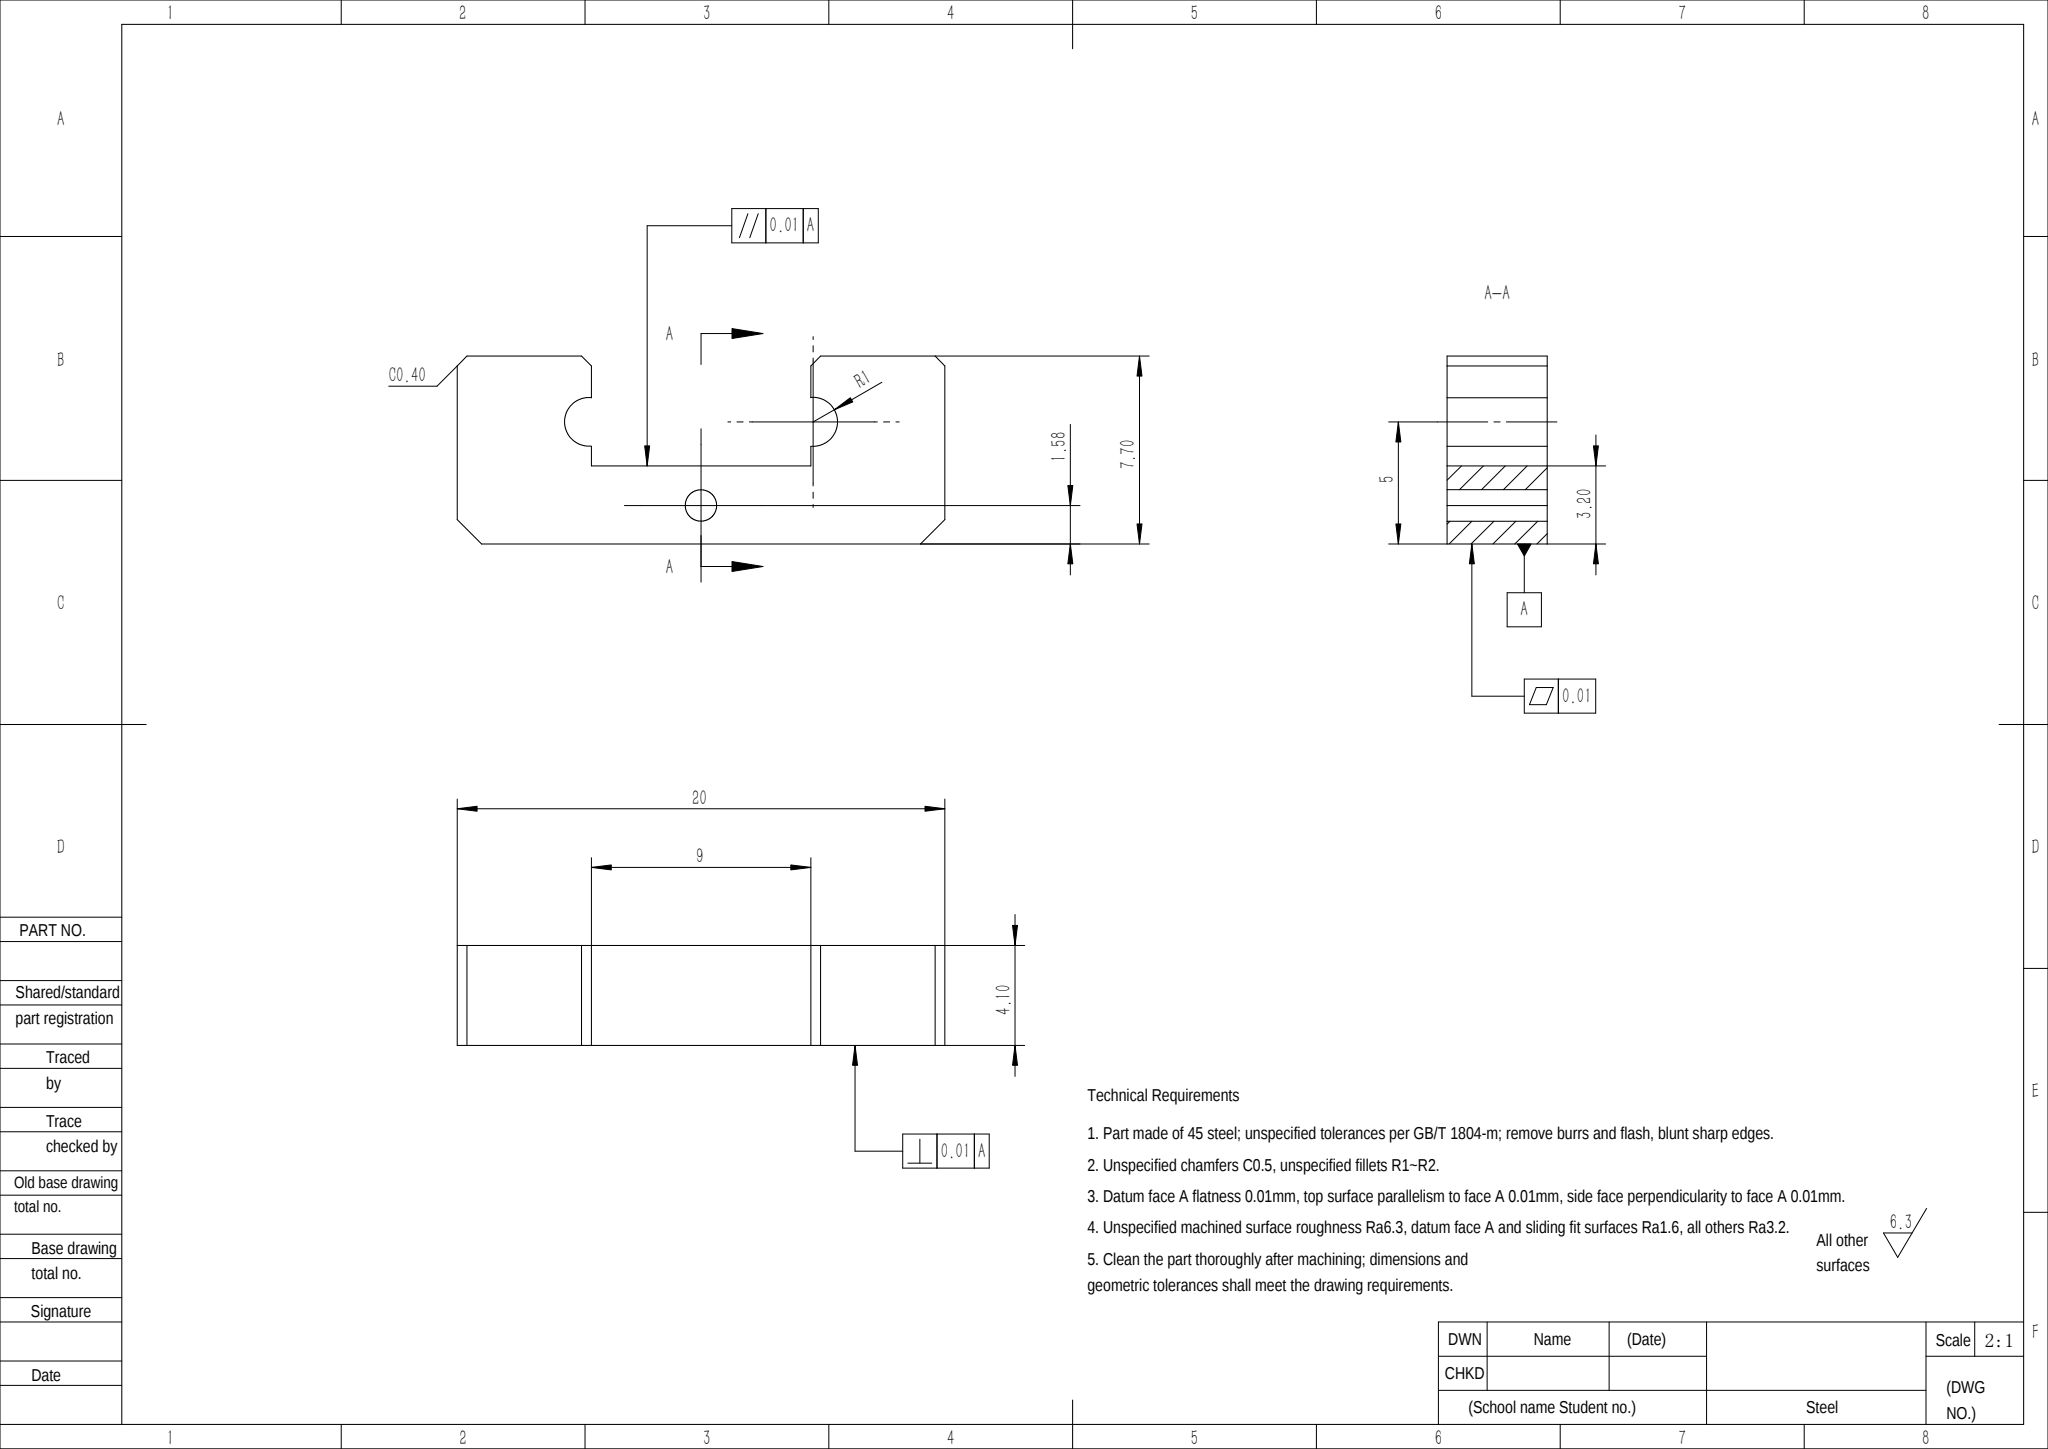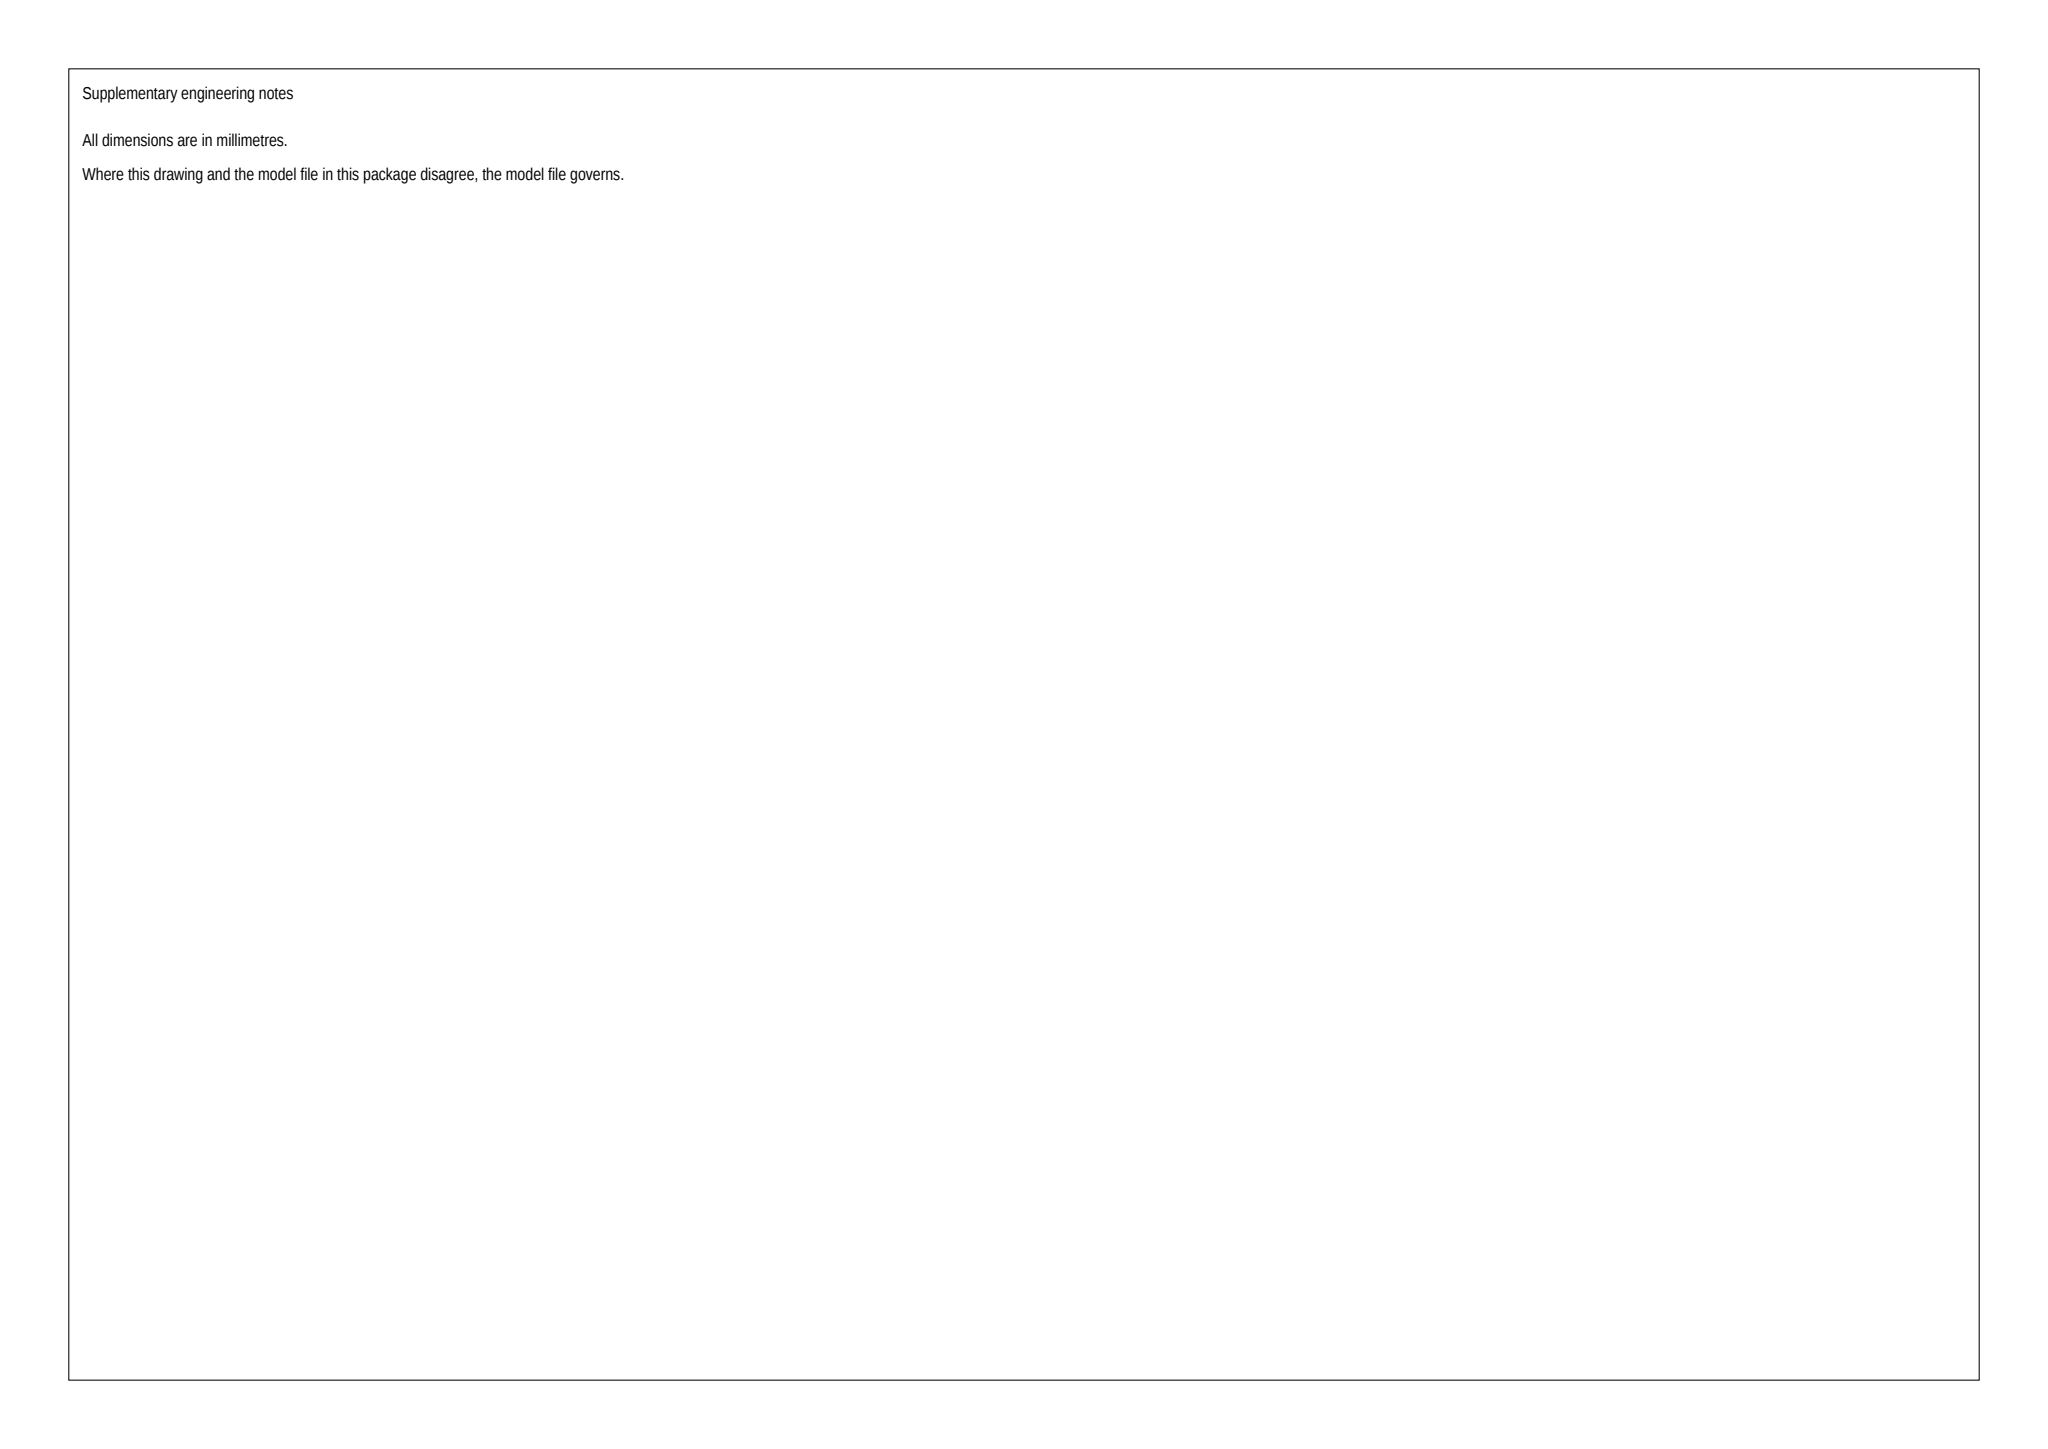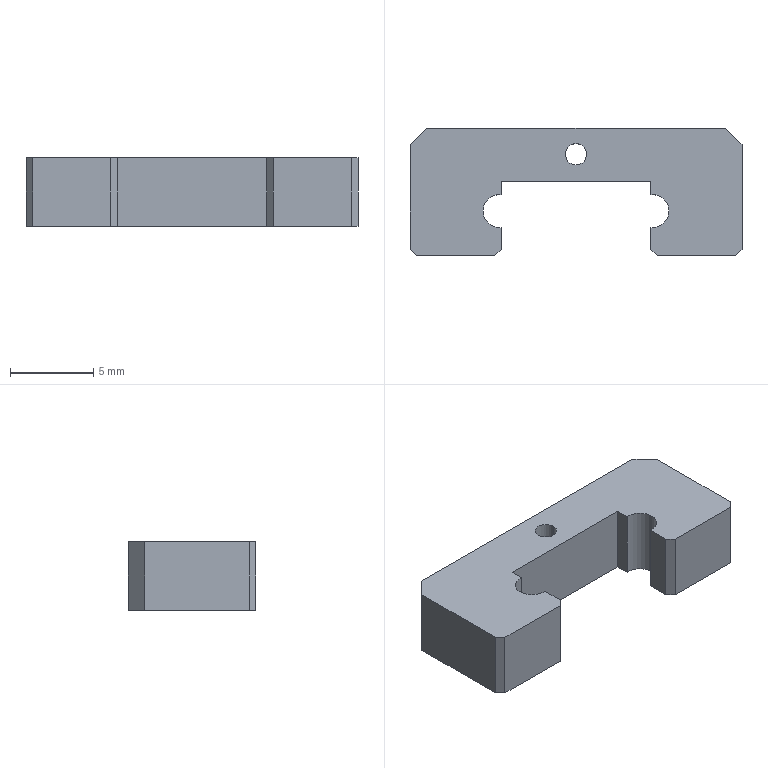Part | SolidWorks | mm | material 45 steel | 1 solid | 22 faces | box 20 x 7.7 x 4.1 mm | volume 440 mm3 | plane 18 | cylinder 4 | commonest cylinder face diameters 1.288 x2 2 x2
STEP:
#1=CARTESIAN_POINT('',(0.644,2.123,-14.95));
#2=VERTEX_POINT('',#1);
#3=CARTESIAN_POINT('',(-0.644,2.123,-14.95));
#4=VERTEX_POINT('',#3);
#5=CARTESIAN_POINT('',(0.,2.123,-14.95));
#6=DIRECTION('',(0.,0.,1.));
#7=DIRECTION('',(1.,0.,0.));
#8=AXIS2_PLACEMENT_3D('',#5,#6,#7);
#9=CIRCLE('',#8,0.644);
#10=EDGE_CURVE('',#2,#4,#9,.T.);
#11=ORIENTED_EDGE('',*,*,#10,.T.);
#12=CARTESIAN_POINT('',(-0.644,2.123,-19.05));
#13=VERTEX_POINT('',#12);
#14=CARTESIAN_POINT('',(-0.644,2.123,-19.05));
#15=CARTESIAN_POINT('',(-0.644,2.123,-17.683));
#16=CARTESIAN_POINT('',(-0.644,2.123,-16.317));
#17=CARTESIAN_POINT('',(-0.644,2.123,-14.95));
#18=B_SPLINE_CURVE_WITH_KNOTS('',3,(#14,#15,#16,#17),.UNSPECIFIED.,.F.,.F.,(4,4),(0.,4.1),.UNSPECIFIED.);
#19=EDGE_CURVE('',#13,#4,#18,.T.);
#20=ORIENTED_EDGE('',*,*,#19,.F.);
#21=CARTESIAN_POINT('',(0.644,2.123,-19.05));
#22=VERTEX_POINT('',#21);
#23=CARTESIAN_POINT('',(0.,2.123,-19.05));
#24=DIRECTION('',(0.,0.,1.));
#25=DIRECTION('',(1.,0.,0.));
#26=AXIS2_PLACEMENT_3D('',#23,#24,#25);
#27=CIRCLE('',#26,0.644);
#28=EDGE_CURVE('',#22,#13,#27,.T.);
#29=ORIENTED_EDGE('',*,*,#28,.F.);
#30=CARTESIAN_POINT('',(0.644,2.123,-19.05));
#31=DIRECTION('',(0.,0.,1.));
#32=VECTOR('',#31,1000.);
#33=LINE('',#30,#32);
#34=EDGE_CURVE('',#22,#2,#33,.T.);
#35=ORIENTED_EDGE('',*,*,#34,.T.);
#36=EDGE_LOOP('',(#11,#20,#29,#35));
#37=FACE_OUTER_BOUND('',#36,.T.);
#38=CARTESIAN_POINT('',(0.,2.123,-19.05));
#39=DIRECTION('',(0.,0.,1.));
#40=DIRECTION('',(-0.,-1.,0.));
#41=AXIS2_PLACEMENT_3D('',#38,#39,#40);
#42=CYLINDRICAL_SURFACE('',#41,0.644);
#43=ADVANCED_FACE('',(#37),#42,.F.);
#44=CARTESIAN_POINT('',(0.,2.123,-19.05));
#45=DIRECTION('',(0.,0.,1.));
#46=DIRECTION('',(1.,0.,0.));
#47=AXIS2_PLACEMENT_3D('',#44,#45,#46);
#48=CIRCLE('',#47,0.644);
#49=EDGE_CURVE('',#13,#22,#48,.T.);
#50=ORIENTED_EDGE('',*,*,#49,.F.);
#51=ORIENTED_EDGE('',*,*,#19,.T.);
#52=CARTESIAN_POINT('',(0.,2.123,-14.95));
#53=DIRECTION('',(0.,0.,1.));
#54=DIRECTION('',(1.,0.,0.));
#55=AXIS2_PLACEMENT_3D('',#52,#53,#54);
#56=CIRCLE('',#55,0.644);
#57=EDGE_CURVE('',#4,#2,#56,.T.);
#58=ORIENTED_EDGE('',*,*,#57,.T.);
#59=ORIENTED_EDGE('',*,*,#34,.F.);
#60=EDGE_LOOP('',(#50,#51,#58,#59));
#61=FACE_OUTER_BOUND('',#60,.T.);
#62=CARTESIAN_POINT('',(0.,2.123,-19.05));
#63=DIRECTION('',(0.,0.,1.));
#64=DIRECTION('',(-0.,1.,0.));
#65=AXIS2_PLACEMENT_3D('',#62,#63,#64);
#66=CYLINDRICAL_SURFACE('',#65,0.644);
#67=ADVANCED_FACE('',(#61),#66,.F.);
#68=CARTESIAN_POINT('',(-9.6,-4.,-14.95));
#69=VERTEX_POINT('',#68);
#70=CARTESIAN_POINT('',(-4.9,-4.,-14.95));
#71=VERTEX_POINT('',#70);
#72=CARTESIAN_POINT('',(0.,-4.,-14.95));
#73=DIRECTION('',(1.,0.,0.));
#74=VECTOR('',#73,1000.);
#75=LINE('',#72,#74);
#76=EDGE_CURVE('',#69,#71,#75,.T.);
#77=ORIENTED_EDGE('',*,*,#76,.T.);
#78=CARTESIAN_POINT('',(-4.5,-3.6,-14.95));
#79=VERTEX_POINT('',#78);
#80=CARTESIAN_POINT('',(-4.5,-3.6,-14.95));
#81=DIRECTION('',(-0.7071,-0.7071,0.));
#82=VECTOR('',#81,1000.);
#83=LINE('',#80,#82);
#84=EDGE_CURVE('',#79,#71,#83,.T.);
#85=ORIENTED_EDGE('',*,*,#84,.F.);
#86=CARTESIAN_POINT('',(-4.5,-2.295,-14.95));
#87=VERTEX_POINT('',#86);
#88=CARTESIAN_POINT('',(-4.5,0.,-14.95));
#89=DIRECTION('',(0.,1.,0.));
#90=VECTOR('',#89,1000.);
#91=LINE('',#88,#90);
#92=EDGE_CURVE('',#79,#87,#91,.T.);
#93=ORIENTED_EDGE('',*,*,#92,.T.);
#94=CARTESIAN_POINT('',(-4.5,-0.305,-14.95));
#95=VERTEX_POINT('',#94);
#96=CARTESIAN_POINT('',(-4.6,-1.3,-14.95));
#97=DIRECTION('',(0.,0.,1.));
#98=DIRECTION('',(1.,0.,0.));
#99=AXIS2_PLACEMENT_3D('',#96,#97,#98);
#100=CIRCLE('',#99,1.);
#101=EDGE_CURVE('',#95,#87,#100,.T.);
#102=ORIENTED_EDGE('',*,*,#101,.F.);
#103=CARTESIAN_POINT('',(-4.5,0.5,-14.95));
#104=VERTEX_POINT('',#103);
#105=CARTESIAN_POINT('',(-4.5,-0.,-14.95));
#106=DIRECTION('',(-0.,1.,0.));
#107=VECTOR('',#106,1000.);
#108=LINE('',#105,#107);
#109=EDGE_CURVE('',#95,#104,#108,.T.);
#110=ORIENTED_EDGE('',*,*,#109,.T.);
#111=CARTESIAN_POINT('',(4.5,0.5,-14.95));
#112=VERTEX_POINT('',#111);
#113=CARTESIAN_POINT('',(0.,0.5,-14.95));
#114=DIRECTION('',(1.,0.,0.));
#115=VECTOR('',#114,1000.);
#116=LINE('',#113,#115);
#117=EDGE_CURVE('',#104,#112,#116,.T.);
#118=ORIENTED_EDGE('',*,*,#117,.T.);
#119=CARTESIAN_POINT('',(4.5,-0.305,-14.95));
#120=VERTEX_POINT('',#119);
#121=CARTESIAN_POINT('',(4.5,0.,-14.95));
#122=DIRECTION('',(-0.,1.,0.));
#123=VECTOR('',#122,1000.);
#124=LINE('',#121,#123);
#125=EDGE_CURVE('',#120,#112,#124,.T.);
#126=ORIENTED_EDGE('',*,*,#125,.F.);
#127=CARTESIAN_POINT('',(4.5,-2.295,-14.95));
#128=VERTEX_POINT('',#127);
#129=CARTESIAN_POINT('',(4.6,-1.3,-14.95));
#130=DIRECTION('',(0.,0.,1.));
#131=DIRECTION('',(1.,0.,0.));
#132=AXIS2_PLACEMENT_3D('',#129,#130,#131);
#133=CIRCLE('',#132,1.);
#134=EDGE_CURVE('',#128,#120,#133,.T.);
#135=ORIENTED_EDGE('',*,*,#134,.F.);
#136=CARTESIAN_POINT('',(4.5,-3.6,-14.95));
#137=VERTEX_POINT('',#136);
#138=CARTESIAN_POINT('',(4.5,0.,-14.95));
#139=DIRECTION('',(0.,1.,0.));
#140=VECTOR('',#139,1000.);
#141=LINE('',#138,#140);
#142=EDGE_CURVE('',#137,#128,#141,.T.);
#143=ORIENTED_EDGE('',*,*,#142,.F.);
#144=CARTESIAN_POINT('',(4.9,-4.,-14.95));
#145=VERTEX_POINT('',#144);
#146=CARTESIAN_POINT('',(4.9,-4.,-14.95));
#147=DIRECTION('',(-0.7071,0.7071,0.));
#148=VECTOR('',#147,1000.);
#149=LINE('',#146,#148);
#150=EDGE_CURVE('',#145,#137,#149,.T.);
#151=ORIENTED_EDGE('',*,*,#150,.F.);
#152=CARTESIAN_POINT('',(9.6,-4.,-14.95));
#153=VERTEX_POINT('',#152);
#154=CARTESIAN_POINT('',(0.,-4.,-14.95));
#155=DIRECTION('',(1.,0.,0.));
#156=VECTOR('',#155,1000.);
#157=LINE('',#154,#156);
#158=EDGE_CURVE('',#145,#153,#157,.T.);
#159=ORIENTED_EDGE('',*,*,#158,.T.);
#160=CARTESIAN_POINT('',(10.,-3.6,-14.95));
#161=VERTEX_POINT('',#160);
#162=CARTESIAN_POINT('',(10.,-3.6,-14.95));
#163=DIRECTION('',(-0.7071,-0.7071,0.));
#164=VECTOR('',#163,1000.);
#165=LINE('',#162,#164);
#166=EDGE_CURVE('',#161,#153,#165,.T.);
#167=ORIENTED_EDGE('',*,*,#166,.F.);
#168=CARTESIAN_POINT('',(10.,2.7,-14.95));
#169=VERTEX_POINT('',#168);
#170=CARTESIAN_POINT('',(10.,-0.,-14.95));
#171=DIRECTION('',(0.,1.,0.));
#172=VECTOR('',#171,1000.);
#173=LINE('',#170,#172);
#174=EDGE_CURVE('',#161,#169,#173,.T.);
#175=ORIENTED_EDGE('',*,*,#174,.T.);
#176=CARTESIAN_POINT('',(9.,3.7,-14.95));
#177=VERTEX_POINT('',#176);
#178=CARTESIAN_POINT('',(9.,3.7,-14.95));
#179=DIRECTION('',(0.7071,-0.7071,0.));
#180=VECTOR('',#179,1000.);
#181=LINE('',#178,#180);
#182=EDGE_CURVE('',#177,#169,#181,.T.);
#183=ORIENTED_EDGE('',*,*,#182,.F.);
#184=CARTESIAN_POINT('',(-9.,3.7,-14.95));
#185=VERTEX_POINT('',#184);
#186=CARTESIAN_POINT('',(0.,3.7,-14.95));
#187=DIRECTION('',(1.,-0.,0.));
#188=VECTOR('',#187,1000.);
#189=LINE('',#186,#188);
#190=EDGE_CURVE('',#185,#177,#189,.T.);
#191=ORIENTED_EDGE('',*,*,#190,.F.);
#192=CARTESIAN_POINT('',(-10.,2.7,-14.95));
#193=VERTEX_POINT('',#192);
#194=CARTESIAN_POINT('',(-10.,2.7,-14.95));
#195=DIRECTION('',(0.7071,0.7071,0.));
#196=VECTOR('',#195,1000.);
#197=LINE('',#194,#196);
#198=EDGE_CURVE('',#193,#185,#197,.T.);
#199=ORIENTED_EDGE('',*,*,#198,.F.);
#200=CARTESIAN_POINT('',(-10.,-3.6,-14.95));
#201=VERTEX_POINT('',#200);
#202=CARTESIAN_POINT('',(-10.,-0.,-14.95));
#203=DIRECTION('',(-0.,1.,0.));
#204=VECTOR('',#203,1000.);
#205=LINE('',#202,#204);
#206=EDGE_CURVE('',#201,#193,#205,.T.);
#207=ORIENTED_EDGE('',*,*,#206,.F.);
#208=CARTESIAN_POINT('',(-9.6,-4.,-14.95));
#209=DIRECTION('',(-0.7071,0.7071,0.));
#210=VECTOR('',#209,1000.);
#211=LINE('',#208,#210);
#212=EDGE_CURVE('',#69,#201,#211,.T.);
#213=ORIENTED_EDGE('',*,*,#212,.F.);
#214=EDGE_LOOP('',(#77,#85,#93,#102,#110,#118,#126,#135,#143,#151,#159,#167,#175,#183,#191,#199,#207,#213));
#215=FACE_OUTER_BOUND('',#214,.T.);
#216=ORIENTED_EDGE('',*,*,#10,.F.);
#217=ORIENTED_EDGE('',*,*,#57,.F.);
#218=EDGE_LOOP('',(#216,#217));
#219=FACE_BOUND('',#218,.T.);
#220=CARTESIAN_POINT('',(0.,0.,-14.95));
#221=DIRECTION('',(0.,0.,-1.));
#222=DIRECTION('',(1.,0.,0.));
#223=AXIS2_PLACEMENT_3D('',#220,#221,#222);
#224=PLANE('',#223);
#225=ADVANCED_FACE('',(#215,#219),#224,.F.);
#226=CARTESIAN_POINT('',(-10.,-3.6,-19.05));
#227=VERTEX_POINT('',#226);
#228=CARTESIAN_POINT('',(-9.6,-4.,-19.05));
#229=VERTEX_POINT('',#228);
#230=CARTESIAN_POINT('',(-6.8,-6.8,-19.05));
#231=DIRECTION('',(0.7071,-0.7071,0.));
#232=VECTOR('',#231,1000.);
#233=LINE('',#230,#232);
#234=EDGE_CURVE('',#227,#229,#233,.T.);
#235=ORIENTED_EDGE('',*,*,#234,.T.);
#236=CARTESIAN_POINT('',(-9.6,-4.,-14.95));
#237=DIRECTION('',(0.,0.,1.));
#238=VECTOR('',#237,1000.);
#239=LINE('',#236,#238);
#240=EDGE_CURVE('',#229,#69,#239,.T.);
#241=ORIENTED_EDGE('',*,*,#240,.T.);
#242=ORIENTED_EDGE('',*,*,#212,.T.);
#243=CARTESIAN_POINT('',(-10.,-3.6,-19.05));
#244=DIRECTION('',(0.,0.,-1.));
#245=VECTOR('',#244,1000.);
#246=LINE('',#243,#245);
#247=EDGE_CURVE('',#201,#227,#246,.T.);
#248=ORIENTED_EDGE('',*,*,#247,.T.);
#249=EDGE_LOOP('',(#235,#241,#242,#248));
#250=FACE_OUTER_BOUND('',#249,.T.);
#251=CARTESIAN_POINT('',(-9.6,-4.,-19.05));
#252=DIRECTION('',(-0.7071,-0.7071,0.));
#253=DIRECTION('',(0.,0.,-1.));
#254=AXIS2_PLACEMENT_3D('',#251,#252,#253);
#255=PLANE('',#254);
#256=ADVANCED_FACE('',(#250),#255,.T.);
#257=ORIENTED_EDGE('',*,*,#206,.T.);
#258=CARTESIAN_POINT('',(-10.,2.7,-19.05));
#259=VERTEX_POINT('',#258);
#260=CARTESIAN_POINT('',(-10.,2.7,-19.05));
#261=DIRECTION('',(0.,0.,1.));
#262=VECTOR('',#261,1000.);
#263=LINE('',#260,#262);
#264=EDGE_CURVE('',#259,#193,#263,.T.);
#265=ORIENTED_EDGE('',*,*,#264,.F.);
#266=CARTESIAN_POINT('',(-10.,-0.,-19.05));
#267=DIRECTION('',(-0.,1.,0.));
#268=VECTOR('',#267,1000.);
#269=LINE('',#266,#268);
#270=EDGE_CURVE('',#227,#259,#269,.T.);
#271=ORIENTED_EDGE('',*,*,#270,.F.);
#272=ORIENTED_EDGE('',*,*,#247,.F.);
#273=EDGE_LOOP('',(#257,#265,#271,#272));
#274=FACE_OUTER_BOUND('',#273,.T.);
#275=CARTESIAN_POINT('',(-10.,-0.,-19.05));
#276=DIRECTION('',(-1.,-0.,0.));
#277=DIRECTION('',(0.,-1.,0.));
#278=AXIS2_PLACEMENT_3D('',#275,#276,#277);
#279=PLANE('',#278);
#280=ADVANCED_FACE('',(#274),#279,.T.);
#281=ORIENTED_EDGE('',*,*,#270,.T.);
#282=CARTESIAN_POINT('',(-9.,3.7,-19.05));
#283=VERTEX_POINT('',#282);
#284=CARTESIAN_POINT('',(-6.35,6.35,-19.05));
#285=DIRECTION('',(-0.7071,-0.7071,0.));
#286=VECTOR('',#285,1000.);
#287=LINE('',#284,#286);
#288=EDGE_CURVE('',#283,#259,#287,.T.);
#289=ORIENTED_EDGE('',*,*,#288,.F.);
#290=CARTESIAN_POINT('',(9.,3.7,-19.05));
#291=VERTEX_POINT('',#290);
#292=CARTESIAN_POINT('',(0.,3.7,-19.05));
#293=DIRECTION('',(1.,-0.,0.));
#294=VECTOR('',#293,1000.);
#295=LINE('',#292,#294);
#296=EDGE_CURVE('',#283,#291,#295,.T.);
#297=ORIENTED_EDGE('',*,*,#296,.T.);
#298=CARTESIAN_POINT('',(10.,2.7,-19.05));
#299=VERTEX_POINT('',#298);
#300=CARTESIAN_POINT('',(6.35,6.35,-19.05));
#301=DIRECTION('',(-0.7071,0.7071,0.));
#302=VECTOR('',#301,1000.);
#303=LINE('',#300,#302);
#304=EDGE_CURVE('',#299,#291,#303,.T.);
#305=ORIENTED_EDGE('',*,*,#304,.F.);
#306=CARTESIAN_POINT('',(10.,-3.6,-19.05));
#307=VERTEX_POINT('',#306);
#308=CARTESIAN_POINT('',(10.,-0.,-19.05));
#309=DIRECTION('',(0.,1.,0.));
#310=VECTOR('',#309,1000.);
#311=LINE('',#308,#310);
#312=EDGE_CURVE('',#307,#299,#311,.T.);
#313=ORIENTED_EDGE('',*,*,#312,.F.);
#314=CARTESIAN_POINT('',(9.6,-4.,-19.05));
#315=VERTEX_POINT('',#314);
#316=CARTESIAN_POINT('',(6.8,-6.8,-19.05));
#317=DIRECTION('',(0.7071,0.7071,0.));
#318=VECTOR('',#317,1000.);
#319=LINE('',#316,#318);
#320=EDGE_CURVE('',#315,#307,#319,.T.);
#321=ORIENTED_EDGE('',*,*,#320,.F.);
#322=CARTESIAN_POINT('',(4.9,-4.,-19.05));
#323=VERTEX_POINT('',#322);
#324=CARTESIAN_POINT('',(0.,-4.,-19.05));
#325=DIRECTION('',(1.,0.,0.));
#326=VECTOR('',#325,1000.);
#327=LINE('',#324,#326);
#328=EDGE_CURVE('',#323,#315,#327,.T.);
#329=ORIENTED_EDGE('',*,*,#328,.F.);
#330=CARTESIAN_POINT('',(4.5,-3.6,-19.05));
#331=VERTEX_POINT('',#330);
#332=CARTESIAN_POINT('',(0.45,0.45,-19.05));
#333=DIRECTION('',(0.7071,-0.7071,0.));
#334=VECTOR('',#333,1000.);
#335=LINE('',#332,#334);
#336=EDGE_CURVE('',#331,#323,#335,.T.);
#337=ORIENTED_EDGE('',*,*,#336,.F.);
#338=CARTESIAN_POINT('',(4.5,-2.295,-19.05));
#339=VERTEX_POINT('',#338);
#340=CARTESIAN_POINT('',(4.5,0.,-19.05));
#341=DIRECTION('',(0.,1.,0.));
#342=VECTOR('',#341,1000.);
#343=LINE('',#340,#342);
#344=EDGE_CURVE('',#331,#339,#343,.T.);
#345=ORIENTED_EDGE('',*,*,#344,.T.);
#346=CARTESIAN_POINT('',(4.5,-0.305,-19.05));
#347=VERTEX_POINT('',#346);
#348=CARTESIAN_POINT('',(4.6,-1.3,-19.05));
#349=DIRECTION('',(0.,0.,1.));
#350=DIRECTION('',(1.,0.,0.));
#351=AXIS2_PLACEMENT_3D('',#348,#349,#350);
#352=CIRCLE('',#351,1.);
#353=EDGE_CURVE('',#339,#347,#352,.T.);
#354=ORIENTED_EDGE('',*,*,#353,.T.);
#355=CARTESIAN_POINT('',(4.5,0.5,-19.05));
#356=VERTEX_POINT('',#355);
#357=CARTESIAN_POINT('',(4.5,0.,-19.05));
#358=DIRECTION('',(-0.,1.,0.));
#359=VECTOR('',#358,1000.);
#360=LINE('',#357,#359);
#361=EDGE_CURVE('',#347,#356,#360,.T.);
#362=ORIENTED_EDGE('',*,*,#361,.T.);
#363=CARTESIAN_POINT('',(-4.5,0.5,-19.05));
#364=VERTEX_POINT('',#363);
#365=CARTESIAN_POINT('',(0.,0.5,-19.05));
#366=DIRECTION('',(1.,0.,0.));
#367=VECTOR('',#366,1000.);
#368=LINE('',#365,#367);
#369=EDGE_CURVE('',#364,#356,#368,.T.);
#370=ORIENTED_EDGE('',*,*,#369,.F.);
#371=CARTESIAN_POINT('',(-4.5,-0.305,-19.05));
#372=VERTEX_POINT('',#371);
#373=CARTESIAN_POINT('',(-4.5,-0.,-19.05));
#374=DIRECTION('',(-0.,1.,0.));
#375=VECTOR('',#374,1000.);
#376=LINE('',#373,#375);
#377=EDGE_CURVE('',#372,#364,#376,.T.);
#378=ORIENTED_EDGE('',*,*,#377,.F.);
#379=CARTESIAN_POINT('',(-4.5,-2.295,-19.05));
#380=VERTEX_POINT('',#379);
#381=CARTESIAN_POINT('',(-4.6,-1.3,-19.05));
#382=DIRECTION('',(0.,0.,1.));
#383=DIRECTION('',(1.,0.,0.));
#384=AXIS2_PLACEMENT_3D('',#381,#382,#383);
#385=CIRCLE('',#384,1.);
#386=EDGE_CURVE('',#372,#380,#385,.T.);
#387=ORIENTED_EDGE('',*,*,#386,.T.);
#388=CARTESIAN_POINT('',(-4.5,-3.6,-19.05));
#389=VERTEX_POINT('',#388);
#390=CARTESIAN_POINT('',(-4.5,0.,-19.05));
#391=DIRECTION('',(0.,1.,0.));
#392=VECTOR('',#391,1000.);
#393=LINE('',#390,#392);
#394=EDGE_CURVE('',#389,#380,#393,.T.);
#395=ORIENTED_EDGE('',*,*,#394,.F.);
#396=CARTESIAN_POINT('',(-4.9,-4.,-19.05));
#397=VERTEX_POINT('',#396);
#398=CARTESIAN_POINT('',(-0.45,0.45,-19.05));
#399=DIRECTION('',(0.7071,0.7071,0.));
#400=VECTOR('',#399,1000.);
#401=LINE('',#398,#400);
#402=EDGE_CURVE('',#397,#389,#401,.T.);
#403=ORIENTED_EDGE('',*,*,#402,.F.);
#404=CARTESIAN_POINT('',(0.,-4.,-19.05));
#405=DIRECTION('',(1.,0.,0.));
#406=VECTOR('',#405,1000.);
#407=LINE('',#404,#406);
#408=EDGE_CURVE('',#229,#397,#407,.T.);
#409=ORIENTED_EDGE('',*,*,#408,.F.);
#410=ORIENTED_EDGE('',*,*,#234,.F.);
#411=EDGE_LOOP('',(#281,#289,#297,#305,#313,#321,#329,#337,#345,#354,#362,#370,#378,#387,#395,#403,#409,#410));
#412=FACE_OUTER_BOUND('',#411,.T.);
#413=ORIENTED_EDGE('',*,*,#28,.T.);
#414=ORIENTED_EDGE('',*,*,#49,.T.);
#415=EDGE_LOOP('',(#413,#414));
#416=FACE_BOUND('',#415,.T.);
#417=CARTESIAN_POINT('',(0.,0.,-19.05));
#418=DIRECTION('',(0.,0.,-1.));
#419=DIRECTION('',(1.,0.,0.));
#420=AXIS2_PLACEMENT_3D('',#417,#418,#419);
#421=PLANE('',#420);
#422=ADVANCED_FACE('',(#412,#416),#421,.T.);
#423=ORIENTED_EDGE('',*,*,#408,.T.);
#424=CARTESIAN_POINT('',(-4.9,-4.,-19.05));
#425=DIRECTION('',(0.,0.,-1.));
#426=VECTOR('',#425,1000.);
#427=LINE('',#424,#426);
#428=EDGE_CURVE('',#71,#397,#427,.T.);
#429=ORIENTED_EDGE('',*,*,#428,.F.);
#430=ORIENTED_EDGE('',*,*,#76,.F.);
#431=ORIENTED_EDGE('',*,*,#240,.F.);
#432=EDGE_LOOP('',(#423,#429,#430,#431));
#433=FACE_OUTER_BOUND('',#432,.T.);
#434=CARTESIAN_POINT('',(0.,-4.,-19.05));
#435=DIRECTION('',(0.,1.,0.));
#436=DIRECTION('',(0.,0.,-1.));
#437=AXIS2_PLACEMENT_3D('',#434,#435,#436);
#438=PLANE('',#437);
#439=ADVANCED_FACE('',(#433),#438,.F.);
#440=ORIENTED_EDGE('',*,*,#402,.T.);
#441=CARTESIAN_POINT('',(-4.5,-3.6,-19.05));
#442=DIRECTION('',(0.,0.,1.));
#443=VECTOR('',#442,1000.);
#444=LINE('',#441,#443);
#445=EDGE_CURVE('',#389,#79,#444,.T.);
#446=ORIENTED_EDGE('',*,*,#445,.T.);
#447=ORIENTED_EDGE('',*,*,#84,.T.);
#448=ORIENTED_EDGE('',*,*,#428,.T.);
#449=EDGE_LOOP('',(#440,#446,#447,#448));
#450=FACE_OUTER_BOUND('',#449,.T.);
#451=CARTESIAN_POINT('',(-4.5,-3.6,-19.05));
#452=DIRECTION('',(-0.7071,0.7071,0.));
#453=DIRECTION('',(0.,0.,1.));
#454=AXIS2_PLACEMENT_3D('',#451,#452,#453);
#455=PLANE('',#454);
#456=ADVANCED_FACE('',(#450),#455,.F.);
#457=ORIENTED_EDGE('',*,*,#394,.T.);
#458=CARTESIAN_POINT('',(-4.5,-2.295,-19.05));
#459=DIRECTION('',(0.,0.,1.));
#460=VECTOR('',#459,1000.);
#461=LINE('',#458,#460);
#462=EDGE_CURVE('',#380,#87,#461,.T.);
#463=ORIENTED_EDGE('',*,*,#462,.T.);
#464=ORIENTED_EDGE('',*,*,#92,.F.);
#465=ORIENTED_EDGE('',*,*,#445,.F.);
#466=EDGE_LOOP('',(#457,#463,#464,#465));
#467=FACE_OUTER_BOUND('',#466,.T.);
#468=CARTESIAN_POINT('',(-4.5,0.,-19.05));
#469=DIRECTION('',(-1.,0.,0.));
#470=DIRECTION('',(-0.,-1.,0.));
#471=AXIS2_PLACEMENT_3D('',#468,#469,#470);
#472=PLANE('',#471);
#473=ADVANCED_FACE('',(#467),#472,.F.);
#474=ORIENTED_EDGE('',*,*,#462,.F.);
#475=ORIENTED_EDGE('',*,*,#386,.F.);
#476=CARTESIAN_POINT('',(-4.5,-0.305,-19.05));
#477=DIRECTION('',(0.,0.,1.));
#478=VECTOR('',#477,1000.);
#479=LINE('',#476,#478);
#480=EDGE_CURVE('',#372,#95,#479,.T.);
#481=ORIENTED_EDGE('',*,*,#480,.T.);
#482=ORIENTED_EDGE('',*,*,#101,.T.);
#483=EDGE_LOOP('',(#474,#475,#481,#482));
#484=FACE_OUTER_BOUND('',#483,.T.);
#485=CARTESIAN_POINT('',(-4.6,-1.3,-19.05));
#486=DIRECTION('',(0.,0.,1.));
#487=DIRECTION('',(1.,-0.,0.));
#488=AXIS2_PLACEMENT_3D('',#485,#486,#487);
#489=CYLINDRICAL_SURFACE('',#488,1.);
#490=ADVANCED_FACE('',(#484),#489,.F.);
#491=ORIENTED_EDGE('',*,*,#109,.F.);
#492=ORIENTED_EDGE('',*,*,#480,.F.);
#493=ORIENTED_EDGE('',*,*,#377,.T.);
#494=CARTESIAN_POINT('',(-4.5,0.5,-19.05));
#495=DIRECTION('',(0.,0.,1.));
#496=VECTOR('',#495,1000.);
#497=LINE('',#494,#496);
#498=EDGE_CURVE('',#364,#104,#497,.T.);
#499=ORIENTED_EDGE('',*,*,#498,.T.);
#500=EDGE_LOOP('',(#491,#492,#493,#499));
#501=FACE_OUTER_BOUND('',#500,.T.);
#502=CARTESIAN_POINT('',(-4.5,-0.,-19.05));
#503=DIRECTION('',(-1.,-0.,0.));
#504=DIRECTION('',(0.,-1.,0.));
#505=AXIS2_PLACEMENT_3D('',#502,#503,#504);
#506=PLANE('',#505);
#507=ADVANCED_FACE('',(#501),#506,.F.);
#508=ORIENTED_EDGE('',*,*,#117,.F.);
#509=ORIENTED_EDGE('',*,*,#498,.F.);
#510=ORIENTED_EDGE('',*,*,#369,.T.);
#511=CARTESIAN_POINT('',(4.5,0.5,-19.05));
#512=DIRECTION('',(0.,0.,1.));
#513=VECTOR('',#512,1000.);
#514=LINE('',#511,#513);
#515=EDGE_CURVE('',#356,#112,#514,.T.);
#516=ORIENTED_EDGE('',*,*,#515,.T.);
#517=EDGE_LOOP('',(#508,#509,#510,#516));
#518=FACE_OUTER_BOUND('',#517,.T.);
#519=CARTESIAN_POINT('',(0.,0.5,-19.05));
#520=DIRECTION('',(0.,1.,0.));
#521=DIRECTION('',(0.,0.,-1.));
#522=AXIS2_PLACEMENT_3D('',#519,#520,#521);
#523=PLANE('',#522);
#524=ADVANCED_FACE('',(#518),#523,.F.);
#525=ORIENTED_EDGE('',*,*,#125,.T.);
#526=ORIENTED_EDGE('',*,*,#515,.F.);
#527=ORIENTED_EDGE('',*,*,#361,.F.);
#528=CARTESIAN_POINT('',(4.5,-0.305,-19.05));
#529=DIRECTION('',(0.,0.,1.));
#530=VECTOR('',#529,1000.);
#531=LINE('',#528,#530);
#532=EDGE_CURVE('',#347,#120,#531,.T.);
#533=ORIENTED_EDGE('',*,*,#532,.T.);
#534=EDGE_LOOP('',(#525,#526,#527,#533));
#535=FACE_OUTER_BOUND('',#534,.T.);
#536=CARTESIAN_POINT('',(4.5,0.,-19.05));
#537=DIRECTION('',(-1.,-0.,0.));
#538=DIRECTION('',(0.,-1.,0.));
#539=AXIS2_PLACEMENT_3D('',#536,#537,#538);
#540=PLANE('',#539);
#541=ADVANCED_FACE('',(#535),#540,.T.);
#542=CARTESIAN_POINT('',(4.5,-2.295,-19.05));
#543=DIRECTION('',(0.,0.,1.));
#544=VECTOR('',#543,1000.);
#545=LINE('',#542,#544);
#546=EDGE_CURVE('',#339,#128,#545,.T.);
#547=ORIENTED_EDGE('',*,*,#546,.T.);
#548=ORIENTED_EDGE('',*,*,#134,.T.);
#549=ORIENTED_EDGE('',*,*,#532,.F.);
#550=ORIENTED_EDGE('',*,*,#353,.F.);
#551=EDGE_LOOP('',(#547,#548,#549,#550));
#552=FACE_OUTER_BOUND('',#551,.T.);
#553=CARTESIAN_POINT('',(4.6,-1.3,-19.05));
#554=DIRECTION('',(0.,0.,1.));
#555=DIRECTION('',(-1.,0.,0.));
#556=AXIS2_PLACEMENT_3D('',#553,#554,#555);
#557=CYLINDRICAL_SURFACE('',#556,1.);
#558=ADVANCED_FACE('',(#552),#557,.F.);
#559=ORIENTED_EDGE('',*,*,#142,.T.);
#560=ORIENTED_EDGE('',*,*,#546,.F.);
#561=ORIENTED_EDGE('',*,*,#344,.F.);
#562=CARTESIAN_POINT('',(4.5,-3.6,-19.05));
#563=DIRECTION('',(0.,0.,-1.));
#564=VECTOR('',#563,1000.);
#565=LINE('',#562,#564);
#566=EDGE_CURVE('',#137,#331,#565,.T.);
#567=ORIENTED_EDGE('',*,*,#566,.F.);
#568=EDGE_LOOP('',(#559,#560,#561,#567));
#569=FACE_OUTER_BOUND('',#568,.T.);
#570=CARTESIAN_POINT('',(4.5,0.,-19.05));
#571=DIRECTION('',(-1.,0.,0.));
#572=DIRECTION('',(0.,0.,-1.));
#573=AXIS2_PLACEMENT_3D('',#570,#571,#572);
#574=PLANE('',#573);
#575=ADVANCED_FACE('',(#569),#574,.T.);
#576=ORIENTED_EDGE('',*,*,#336,.T.);
#577=CARTESIAN_POINT('',(4.9,-4.,-14.95));
#578=DIRECTION('',(0.,0.,1.));
#579=VECTOR('',#578,1000.);
#580=LINE('',#577,#579);
#581=EDGE_CURVE('',#323,#145,#580,.T.);
#582=ORIENTED_EDGE('',*,*,#581,.T.);
#583=ORIENTED_EDGE('',*,*,#150,.T.);
#584=ORIENTED_EDGE('',*,*,#566,.T.);
#585=EDGE_LOOP('',(#576,#582,#583,#584));
#586=FACE_OUTER_BOUND('',#585,.T.);
#587=CARTESIAN_POINT('',(4.9,-4.,-19.05));
#588=DIRECTION('',(-0.7071,-0.7071,0.));
#589=DIRECTION('',(0.,0.,-1.));
#590=AXIS2_PLACEMENT_3D('',#587,#588,#589);
#591=PLANE('',#590);
#592=ADVANCED_FACE('',(#586),#591,.T.);
#593=ORIENTED_EDGE('',*,*,#328,.T.);
#594=CARTESIAN_POINT('',(9.6,-4.,-19.05));
#595=DIRECTION('',(0.,0.,-1.));
#596=VECTOR('',#595,1000.);
#597=LINE('',#594,#596);
#598=EDGE_CURVE('',#153,#315,#597,.T.);
#599=ORIENTED_EDGE('',*,*,#598,.F.);
#600=ORIENTED_EDGE('',*,*,#158,.F.);
#601=ORIENTED_EDGE('',*,*,#581,.F.);
#602=EDGE_LOOP('',(#593,#599,#600,#601));
#603=FACE_OUTER_BOUND('',#602,.T.);
#604=CARTESIAN_POINT('',(0.,-4.,-19.05));
#605=DIRECTION('',(0.,1.,0.));
#606=DIRECTION('',(0.,0.,-1.));
#607=AXIS2_PLACEMENT_3D('',#604,#605,#606);
#608=PLANE('',#607);
#609=ADVANCED_FACE('',(#603),#608,.F.);
#610=ORIENTED_EDGE('',*,*,#320,.T.);
#611=CARTESIAN_POINT('',(10.,-3.6,-19.05));
#612=DIRECTION('',(0.,0.,1.));
#613=VECTOR('',#612,1000.);
#614=LINE('',#611,#613);
#615=EDGE_CURVE('',#307,#161,#614,.T.);
#616=ORIENTED_EDGE('',*,*,#615,.T.);
#617=ORIENTED_EDGE('',*,*,#166,.T.);
#618=ORIENTED_EDGE('',*,*,#598,.T.);
#619=EDGE_LOOP('',(#610,#616,#617,#618));
#620=FACE_OUTER_BOUND('',#619,.T.);
#621=CARTESIAN_POINT('',(10.,-3.6,-19.05));
#622=DIRECTION('',(-0.7071,0.7071,0.));
#623=DIRECTION('',(0.,0.,1.));
#624=AXIS2_PLACEMENT_3D('',#621,#622,#623);
#625=PLANE('',#624);
#626=ADVANCED_FACE('',(#620),#625,.F.);
#627=ORIENTED_EDGE('',*,*,#312,.T.);
#628=CARTESIAN_POINT('',(10.,2.7,-19.05));
#629=DIRECTION('',(0.,0.,-1.));
#630=VECTOR('',#629,1000.);
#631=LINE('',#628,#630);
#632=EDGE_CURVE('',#169,#299,#631,.T.);
#633=ORIENTED_EDGE('',*,*,#632,.F.);
#634=ORIENTED_EDGE('',*,*,#174,.F.);
#635=ORIENTED_EDGE('',*,*,#615,.F.);
#636=EDGE_LOOP('',(#627,#633,#634,#635));
#637=FACE_OUTER_BOUND('',#636,.T.);
#638=CARTESIAN_POINT('',(10.,-0.,-19.05));
#639=DIRECTION('',(-1.,0.,0.));
#640=DIRECTION('',(-0.,-1.,0.));
#641=AXIS2_PLACEMENT_3D('',#638,#639,#640);
#642=PLANE('',#641);
#643=ADVANCED_FACE('',(#637),#642,.F.);
#644=ORIENTED_EDGE('',*,*,#304,.T.);
#645=CARTESIAN_POINT('',(9.,3.7,-14.95));
#646=DIRECTION('',(0.,0.,1.));
#647=VECTOR('',#646,1000.);
#648=LINE('',#645,#647);
#649=EDGE_CURVE('',#291,#177,#648,.T.);
#650=ORIENTED_EDGE('',*,*,#649,.T.);
#651=ORIENTED_EDGE('',*,*,#182,.T.);
#652=ORIENTED_EDGE('',*,*,#632,.T.);
#653=EDGE_LOOP('',(#644,#650,#651,#652));
#654=FACE_OUTER_BOUND('',#653,.T.);
#655=CARTESIAN_POINT('',(9.,3.7,-19.05));
#656=DIRECTION('',(0.7071,0.7071,0.));
#657=DIRECTION('',(0.,0.,-1.));
#658=AXIS2_PLACEMENT_3D('',#655,#656,#657);
#659=PLANE('',#658);
#660=ADVANCED_FACE('',(#654),#659,.T.);
#661=ORIENTED_EDGE('',*,*,#190,.T.);
#662=ORIENTED_EDGE('',*,*,#649,.F.);
#663=ORIENTED_EDGE('',*,*,#296,.F.);
#664=CARTESIAN_POINT('',(-9.,3.7,-19.05));
#665=DIRECTION('',(0.,0.,-1.));
#666=VECTOR('',#665,1000.);
#667=LINE('',#664,#666);
#668=EDGE_CURVE('',#185,#283,#667,.T.);
#669=ORIENTED_EDGE('',*,*,#668,.F.);
#670=EDGE_LOOP('',(#661,#662,#663,#669));
#671=FACE_OUTER_BOUND('',#670,.T.);
#672=CARTESIAN_POINT('',(0.,3.7,-19.05));
#673=DIRECTION('',(0.,1.,0.));
#674=DIRECTION('',(-1.,0.,0.));
#675=AXIS2_PLACEMENT_3D('',#672,#673,#674);
#676=PLANE('',#675);
#677=ADVANCED_FACE('',(#671),#676,.T.);
#678=ORIENTED_EDGE('',*,*,#288,.T.);
#679=ORIENTED_EDGE('',*,*,#264,.T.);
#680=ORIENTED_EDGE('',*,*,#198,.T.);
#681=ORIENTED_EDGE('',*,*,#668,.T.);
#682=EDGE_LOOP('',(#678,#679,#680,#681));
#683=FACE_OUTER_BOUND('',#682,.T.);
#684=CARTESIAN_POINT('',(-10.,2.7,-19.05));
#685=DIRECTION('',(0.7071,-0.7071,0.));
#686=DIRECTION('',(0.,0.,1.));
#687=AXIS2_PLACEMENT_3D('',#684,#685,#686);
#688=PLANE('',#687);
#689=ADVANCED_FACE('',(#683),#688,.F.);
#690=CLOSED_SHELL('',(#43,#67,#225,#256,#280,#422,#439,#456,#473,#490,#507,#524,#541,#558,#575,#592,#609,#626,#643,#660,#677,#689));
#691=MANIFOLD_SOLID_BREP('',#690);
#692=CARTESIAN_POINT('',(0.,0.,0.));
#693=DIRECTION('',(0.,0.,1.));
#694=DIRECTION('',(1.,0.,0.));
#695=AXIS2_PLACEMENT_3D('',#692,#693,#694);
#696=(LENGTH_UNIT()NAMED_UNIT(*)SI_UNIT(.MILLI.,.METRE.));
#697=UNCERTAINTY_MEASURE_WITH_UNIT(LENGTH_MEASURE(0.00001),#696,'','');
#698=(NAMED_UNIT(*)PLANE_ANGLE_UNIT()SI_UNIT($,.RADIAN.));
#699=(NAMED_UNIT(*)SI_UNIT($,.STERADIAN.)SOLID_ANGLE_UNIT());
#700=(GEOMETRIC_REPRESENTATION_CONTEXT(3)GLOBAL_UNCERTAINTY_ASSIGNED_CONTEXT((#697))GLOBAL_UNIT_ASSIGNED_CONTEXT((#696,#698,#699))REPRESENTATION_CONTEXT('',''));
#701=ADVANCED_BREP_SHAPE_REPRESENTATION('',(#691,#695),#700);